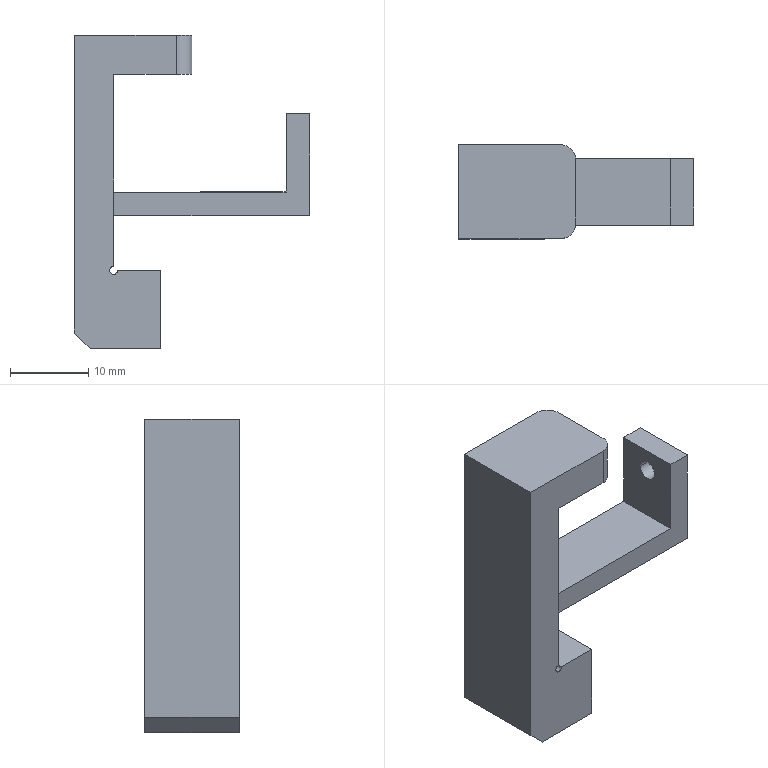Component | SolidWorks | MovingBlock-2 | 1 solid | 24 faces | box 30 x 12 x 40 mm | volume 4558 mm3 | plane 18 | cylinder 6 | commonest cylinder face diameters 2.5 x2 1 x2 4 x2
build123d program:
from build123d import *

# Parameters (mm, degrees)
SKETCH1_W         = 12
SKETCH1_H         = 20
EXTRUDE1_DEPTH    = 5
SKETCH2_W         = 8.5
SKETCH2_H         = 3
EXTRUDE2_DEPTH    = 25
SKETCH3_W         = 12
SKETCH3_H         = 10
EXTRUDE3_DEPTH    = 6
CHAMFER1_SIZE     = 2
SKETCH6_R         = 0.5
EXTRUDE4_DEPTH    = 30.479
SKETCH7_W         = 8.5
SKETCH7_H         = 3
EXTRUDE5_DEPTH    = 10
M3_TAPPED_HOLE1_D = 2.5
SKETCH12_W        = 12
SKETCH12_H        = 5
EXTRUDE8_DEPTH    = 20
SKETCH13_W        = 12
SKETCH13_H        = 5
EXTRUDE9_DEPTH    = 10
FILLET3_R         = 2


with BuildPart() as part:
    # Sketch1 → Extrude1 (new body)
    with BuildSketch(Plane.XY):
        Rectangle(SKETCH1_W, SKETCH1_H)
    extrude(amount=EXTRUDE1_DEPTH)

    # Sketch2 → Extrude2 (add)
    with BuildSketch(Plane(origin=(0, 0, 0), x_dir=(-1, 0, 0), z_dir=(0, 0, -1))):
        with Locations((0, -8.5)):
            Rectangle(SKETCH2_W, SKETCH2_H)
    extrude(amount=EXTRUDE2_DEPTH)

    # Sketch3 → Extrude3 (add)
    with BuildSketch(Plane(origin=(0, 0, 0), x_dir=(-1, 0, 0), z_dir=(0, 0, -1))):
        with Locations((0, 5)):
            Rectangle(SKETCH3_W, SKETCH3_H)
    extrude(amount=EXTRUDE3_DEPTH)

    # Chamfer1
    chamfer1_edges = [part.edges().sort_by_distance(p)[0] for p in [
        (0, 10, 5),
    ]]
    chamfer(chamfer1_edges, length=CHAMFER1_SIZE)

    # Sketch6 → Extrude4 (cut, through all)
    with BuildSketch(Plane.ZY.offset(6)):
        Circle(SKETCH6_R)
    extrude(amount=-EXTRUDE4_DEPTH, mode=Mode.SUBTRACT)

    # Sketch7 → Extrude5 (add)
    with BuildSketch(Plane.XZ.offset(10)):
        with Locations((0, -23.5)):
            Rectangle(SKETCH7_W, SKETCH7_H)
    extrude(amount=EXTRUDE5_DEPTH)

    # M3 Tapped Hole1 (through all)
    with Locations(Plane(origin=(0, 0, -25), x_dir=(-1, 0, 0), z_dir=(0, 0, -1))):
        with Locations((0, -17)):
            Hole(M3_TAPPED_HOLE1_D / 2)

    # Sketch12 → Extrude8 (add)
    with BuildSketch(Plane.XZ.offset(10)):
        with Locations((0, 2.5)):
            Rectangle(SKETCH12_W, SKETCH12_H)
    extrude(amount=EXTRUDE8_DEPTH)

    # Sketch13 → Extrude9 (add)
    with BuildSketch(Plane(origin=(0, 0, 0), x_dir=(-1, 0, 0), z_dir=(0, 0, -1))):
        with Locations((0, -27.5)):
            Rectangle(SKETCH13_W, SKETCH13_H)
    extrude(amount=EXTRUDE9_DEPTH)

    # Fillet3
    fillet3_edges = [part.edges().sort_by_distance(p)[0] for p in [
        (6, -27.5, -10),
        (-6, -27.5, -10),
    ]]
    fillet(fillet3_edges, radius=FILLET3_R)


solid = part.part

# Placed as in the assembly
solid = solid.moved(Location((-89, -31.25, 0), (-90, -90, 0)))
STEP:
#1=CARTESIAN_POINT('',(-2.638,-1.181,0.6693));
#2=VERTEX_POINT('',#1);
#3=CARTESIAN_POINT('',(-2.638,-1.28,0.6693));
#4=VERTEX_POINT('',#3);
#5=CARTESIAN_POINT('',(-2.638,-1.23,0.6693));
#6=DIRECTION('',(1.,0.,0.));
#7=DIRECTION('',(0.,-1.,0.));
#8=AXIS2_PLACEMENT_3D('',#5,#6,#7);
#9=CIRCLE('',#8,0.04921);
#10=EDGE_CURVE('',#2,#4,#9,.T.);
#11=ORIENTED_EDGE('',*,*,#10,.F.);
#12=CARTESIAN_POINT('',(-2.52,-1.181,0.6693));
#13=VERTEX_POINT('',#12);
#14=CARTESIAN_POINT('',(-2.52,-1.181,0.6693));
#15=DIRECTION('',(1.,0.,0.));
#16=VECTOR('',#15,39.37);
#17=LINE('',#14,#16);
#18=EDGE_CURVE('',#2,#13,#17,.T.);
#19=ORIENTED_EDGE('',*,*,#18,.T.);
#20=CARTESIAN_POINT('',(-2.52,-1.28,0.6693));
#21=VERTEX_POINT('',#20);
#22=CARTESIAN_POINT('',(-2.52,-1.23,0.6693));
#23=DIRECTION('',(1.,0.,0.));
#24=DIRECTION('',(0.,-1.,0.));
#25=AXIS2_PLACEMENT_3D('',#22,#23,#24);
#26=CIRCLE('',#25,0.04921);
#27=EDGE_CURVE('',#13,#21,#26,.T.);
#28=ORIENTED_EDGE('',*,*,#27,.T.);
#29=CARTESIAN_POINT('',(-2.52,-1.28,0.6693));
#30=DIRECTION('',(1.,0.,0.));
#31=VECTOR('',#30,39.37);
#32=LINE('',#29,#31);
#33=EDGE_CURVE('',#4,#21,#32,.T.);
#34=ORIENTED_EDGE('',*,*,#33,.F.);
#35=EDGE_LOOP('',(#11,#19,#28,#34));
#36=FACE_OUTER_BOUND('',#35,.T.);
#37=CARTESIAN_POINT('',(-2.52,-1.23,0.6693));
#38=DIRECTION('',(1.,0.,0.));
#39=DIRECTION('',(0.,-1.,0.));
#40=AXIS2_PLACEMENT_3D('',#37,#38,#39);
#41=CYLINDRICAL_SURFACE('',#40,0.04921);
#42=ADVANCED_FACE('',(#36),#41,.F.);
#43=CARTESIAN_POINT('',(-3.524,-0.9941,0.));
#44=VERTEX_POINT('',#43);
#45=CARTESIAN_POINT('',(-3.484,-0.9941,-0.));
#46=VERTEX_POINT('',#45);
#47=CARTESIAN_POINT('',(-3.504,-0.9941,0.));
#48=DIRECTION('',(0.,-1.,0.));
#49=DIRECTION('',(-1.,0.,0.));
#50=AXIS2_PLACEMENT_3D('',#47,#48,#49);
#51=CIRCLE('',#50,0.01969);
#52=EDGE_CURVE('',#44,#46,#51,.T.);
#53=ORIENTED_EDGE('',*,*,#52,.F.);
#54=CARTESIAN_POINT('',(-3.524,-1.467,0.));
#55=VERTEX_POINT('',#54);
#56=CARTESIAN_POINT('',(-3.524,-0.9941,0.));
#57=DIRECTION('',(0.,-1.,0.));
#58=VECTOR('',#57,39.37);
#59=LINE('',#56,#58);
#60=EDGE_CURVE('',#44,#55,#59,.T.);
#61=ORIENTED_EDGE('',*,*,#60,.T.);
#62=CARTESIAN_POINT('',(-3.484,-1.467,-0.));
#63=VERTEX_POINT('',#62);
#64=CARTESIAN_POINT('',(-3.504,-1.467,0.));
#65=DIRECTION('',(0.,-1.,0.));
#66=DIRECTION('',(-1.,0.,0.));
#67=AXIS2_PLACEMENT_3D('',#64,#65,#66);
#68=CIRCLE('',#67,0.01969);
#69=EDGE_CURVE('',#55,#63,#68,.T.);
#70=ORIENTED_EDGE('',*,*,#69,.T.);
#71=CARTESIAN_POINT('',(-3.484,-0.9941,-0.));
#72=DIRECTION('',(0.,-1.,0.));
#73=VECTOR('',#72,39.37);
#74=LINE('',#71,#73);
#75=EDGE_CURVE('',#46,#63,#74,.T.);
#76=ORIENTED_EDGE('',*,*,#75,.F.);
#77=EDGE_LOOP('',(#53,#61,#70,#76));
#78=FACE_OUTER_BOUND('',#77,.T.);
#79=CARTESIAN_POINT('',(-3.504,-0.9941,0.));
#80=DIRECTION('',(0.,-1.,0.));
#81=DIRECTION('',(-1.,0.,0.));
#82=AXIS2_PLACEMENT_3D('',#79,#80,#81);
#83=CYLINDRICAL_SURFACE('',#82,0.01969);
#84=ADVANCED_FACE('',(#78),#83,.F.);
#85=CARTESIAN_POINT('',(-3.504,-1.398,0.3937));
#86=VERTEX_POINT('',#85);
#87=CARTESIAN_POINT('',(-3.504,-1.398,0.2756));
#88=VERTEX_POINT('',#87);
#89=CARTESIAN_POINT('',(-3.504,-1.398,0.3937));
#90=DIRECTION('',(-0.,0.,-1.));
#91=VECTOR('',#90,39.37);
#92=LINE('',#89,#91);
#93=EDGE_CURVE('',#86,#88,#92,.T.);
#94=ORIENTED_EDGE('',*,*,#93,.F.);
#95=CARTESIAN_POINT('',(-3.504,-1.063,0.3937));
#96=VERTEX_POINT('',#95);
#97=CARTESIAN_POINT('',(-3.504,-1.467,0.3937));
#98=DIRECTION('',(0.,1.,-0.));
#99=VECTOR('',#98,39.37);
#100=LINE('',#97,#99);
#101=EDGE_CURVE('',#86,#96,#100,.T.);
#102=ORIENTED_EDGE('',*,*,#101,.T.);
#103=CARTESIAN_POINT('',(-3.504,-1.063,0.2756));
#104=VERTEX_POINT('',#103);
#105=CARTESIAN_POINT('',(-3.504,-1.063,0.3937));
#106=DIRECTION('',(0.,-0.,1.));
#107=VECTOR('',#106,39.37);
#108=LINE('',#105,#107);
#109=EDGE_CURVE('',#104,#96,#108,.T.);
#110=ORIENTED_EDGE('',*,*,#109,.F.);
#111=CARTESIAN_POINT('',(-3.504,-1.063,0.2756));
#112=DIRECTION('',(0.,1.,0.));
#113=VECTOR('',#112,39.37);
#114=LINE('',#111,#113);
#115=EDGE_CURVE('',#88,#104,#114,.T.);
#116=ORIENTED_EDGE('',*,*,#115,.F.);
#117=EDGE_LOOP('',(#94,#102,#110,#116));
#118=FACE_BOUND('',#117,.T.);
#119=CARTESIAN_POINT('',(-3.504,-1.467,0.9843));
#120=VERTEX_POINT('',#119);
#121=CARTESIAN_POINT('',(-3.504,-0.9941,0.9843));
#122=VERTEX_POINT('',#121);
#123=CARTESIAN_POINT('',(-3.504,-0.9941,0.9843));
#124=DIRECTION('',(0.,1.,-0.));
#125=VECTOR('',#124,39.37);
#126=LINE('',#123,#125);
#127=EDGE_CURVE('',#120,#122,#126,.T.);
#128=ORIENTED_EDGE('',*,*,#127,.F.);
#129=CARTESIAN_POINT('',(-3.504,-1.467,0.01969));
#130=VERTEX_POINT('',#129);
#131=CARTESIAN_POINT('',(-3.504,-1.467,0.3937));
#132=DIRECTION('',(0.,-0.,1.));
#133=VECTOR('',#132,39.37);
#134=LINE('',#131,#133);
#135=EDGE_CURVE('',#130,#120,#134,.T.);
#136=ORIENTED_EDGE('',*,*,#135,.F.);
#137=CARTESIAN_POINT('',(-3.504,-0.9941,0.01969));
#138=VERTEX_POINT('',#137);
#139=CARTESIAN_POINT('',(-3.504,-0.9941,0.01969));
#140=DIRECTION('',(0.,1.,-0.));
#141=VECTOR('',#140,39.37);
#142=LINE('',#139,#141);
#143=EDGE_CURVE('',#130,#138,#142,.T.);
#144=ORIENTED_EDGE('',*,*,#143,.T.);
#145=CARTESIAN_POINT('',(-3.504,-0.9941,0.3937));
#146=DIRECTION('',(-0.,0.,-1.));
#147=VECTOR('',#146,39.37);
#148=LINE('',#145,#147);
#149=EDGE_CURVE('',#122,#138,#148,.T.);
#150=ORIENTED_EDGE('',*,*,#149,.F.);
#151=EDGE_LOOP('',(#128,#136,#144,#150));
#152=FACE_OUTER_BOUND('',#151,.T.);
#153=CARTESIAN_POINT('',(-3.504,-1.467,-0.3937));
#154=DIRECTION('',(-1.,-0.,-0.));
#155=DIRECTION('',(0.,1.,-0.));
#156=AXIS2_PLACEMENT_3D('',#153,#154,#155);
#157=PLANE('',#156);
#158=ADVANCED_FACE('',(#118,#152),#157,.F.);
#159=ORIENTED_EDGE('',*,*,#101,.F.);
#160=CARTESIAN_POINT('',(-2.638,-1.398,0.3937));
#161=VERTEX_POINT('',#160);
#162=CARTESIAN_POINT('',(-2.52,-1.398,0.3937));
#163=DIRECTION('',(-1.,0.,-0.));
#164=VECTOR('',#163,39.37);
#165=LINE('',#162,#164);
#166=EDGE_CURVE('',#161,#86,#165,.T.);
#167=ORIENTED_EDGE('',*,*,#166,.F.);
#168=CARTESIAN_POINT('',(-2.638,-1.063,0.3937));
#169=VERTEX_POINT('',#168);
#170=CARTESIAN_POINT('',(-2.638,-1.398,0.3937));
#171=DIRECTION('',(0.,-1.,0.));
#172=VECTOR('',#171,39.37);
#173=LINE('',#170,#172);
#174=EDGE_CURVE('',#169,#161,#173,.T.);
#175=ORIENTED_EDGE('',*,*,#174,.F.);
#176=CARTESIAN_POINT('',(-2.52,-1.063,0.3937));
#177=DIRECTION('',(-1.,0.,-0.));
#178=VECTOR('',#177,39.37);
#179=LINE('',#176,#178);
#180=EDGE_CURVE('',#169,#96,#179,.T.);
#181=ORIENTED_EDGE('',*,*,#180,.T.);
#182=EDGE_LOOP('',(#159,#167,#175,#181));
#183=FACE_OUTER_BOUND('',#182,.T.);
#184=CARTESIAN_POINT('',(-3.701,-0.9941,0.3937));
#185=DIRECTION('',(0.,0.,-1.));
#186=DIRECTION('',(-1.,0.,-0.));
#187=AXIS2_PLACEMENT_3D('',#184,#185,#186);
#188=PLANE('',#187);
#189=ADVANCED_FACE('',(#183),#188,.F.);
#190=CARTESIAN_POINT('',(-3.189,-1.467,0.9843));
#191=VERTEX_POINT('',#190);
#192=CARTESIAN_POINT('',(-3.11,-1.467,0.9843));
#193=DIRECTION('',(-1.,0.,-0.));
#194=VECTOR('',#193,39.37);
#195=LINE('',#192,#194);
#196=EDGE_CURVE('',#191,#120,#195,.T.);
#197=ORIENTED_EDGE('',*,*,#196,.F.);
#198=CARTESIAN_POINT('',(-3.189,-1.467,1.181));
#199=VERTEX_POINT('',#198);
#200=CARTESIAN_POINT('',(-3.189,-1.467,0.3937));
#201=DIRECTION('',(0.,-0.,1.));
#202=VECTOR('',#201,39.37);
#203=LINE('',#200,#202);
#204=EDGE_CURVE('',#191,#199,#203,.T.);
#205=ORIENTED_EDGE('',*,*,#204,.T.);
#206=CARTESIAN_POINT('',(-3.701,-1.467,1.181));
#207=VERTEX_POINT('',#206);
#208=CARTESIAN_POINT('',(-3.701,-1.467,1.181));
#209=DIRECTION('',(1.,0.,0.));
#210=VECTOR('',#209,39.37);
#211=LINE('',#208,#210);
#212=EDGE_CURVE('',#207,#199,#211,.T.);
#213=ORIENTED_EDGE('',*,*,#212,.F.);
#214=CARTESIAN_POINT('',(-3.701,-1.467,-0.315));
#215=VERTEX_POINT('',#214);
#216=CARTESIAN_POINT('',(-3.701,-1.467,0.3937));
#217=DIRECTION('',(0.,-0.,1.));
#218=VECTOR('',#217,39.37);
#219=LINE('',#216,#218);
#220=EDGE_CURVE('',#215,#207,#219,.T.);
#221=ORIENTED_EDGE('',*,*,#220,.F.);
#222=CARTESIAN_POINT('',(-3.622,-1.467,-0.3937));
#223=VERTEX_POINT('',#222);
#224=CARTESIAN_POINT('',(-3.701,-1.467,-0.315));
#225=DIRECTION('',(0.7071,0.,-0.7071));
#226=VECTOR('',#225,39.37);
#227=LINE('',#224,#226);
#228=EDGE_CURVE('',#215,#223,#227,.T.);
#229=ORIENTED_EDGE('',*,*,#228,.T.);
#230=CARTESIAN_POINT('',(-3.268,-1.467,-0.3937));
#231=VERTEX_POINT('',#230);
#232=CARTESIAN_POINT('',(-3.701,-1.467,-0.3937));
#233=DIRECTION('',(1.,0.,0.));
#234=VECTOR('',#233,39.37);
#235=LINE('',#232,#234);
#236=EDGE_CURVE('',#223,#231,#235,.T.);
#237=ORIENTED_EDGE('',*,*,#236,.T.);
#238=CARTESIAN_POINT('',(-3.268,-1.467,-0.));
#239=VERTEX_POINT('',#238);
#240=CARTESIAN_POINT('',(-3.268,-1.467,-0.3937));
#241=DIRECTION('',(-0.,0.,-1.));
#242=VECTOR('',#241,39.37);
#243=LINE('',#240,#242);
#244=EDGE_CURVE('',#239,#231,#243,.T.);
#245=ORIENTED_EDGE('',*,*,#244,.F.);
#246=CARTESIAN_POINT('',(-3.268,-1.467,-0.));
#247=DIRECTION('',(-1.,0.,-0.));
#248=VECTOR('',#247,39.37);
#249=LINE('',#246,#248);
#250=EDGE_CURVE('',#239,#63,#249,.T.);
#251=ORIENTED_EDGE('',*,*,#250,.T.);
#252=ORIENTED_EDGE('',*,*,#69,.F.);
#253=CARTESIAN_POINT('',(-3.504,-1.467,0.));
#254=DIRECTION('',(0.,-1.,0.));
#255=DIRECTION('',(-1.,0.,0.));
#256=AXIS2_PLACEMENT_3D('',#253,#254,#255);
#257=CIRCLE('',#256,0.01969);
#258=EDGE_CURVE('',#130,#55,#257,.T.);
#259=ORIENTED_EDGE('',*,*,#258,.F.);
#260=ORIENTED_EDGE('',*,*,#135,.T.);
#261=EDGE_LOOP('',(#197,#205,#213,#221,#229,#237,#245,#251,#252,#259,#260));
#262=FACE_OUTER_BOUND('',#261,.T.);
#263=CARTESIAN_POINT('',(-3.701,-1.467,0.3937));
#264=DIRECTION('',(0.,1.,-0.));
#265=DIRECTION('',(1.,0.,0.));
#266=AXIS2_PLACEMENT_3D('',#263,#264,#265);
#267=PLANE('',#266);
#268=ADVANCED_FACE('',(#262),#267,.F.);
#269=CARTESIAN_POINT('',(-3.189,-0.9941,1.181));
#270=VERTEX_POINT('',#269);
#271=CARTESIAN_POINT('',(-3.701,-0.9941,1.181));
#272=VERTEX_POINT('',#271);
#273=CARTESIAN_POINT('',(-3.701,-0.9941,1.181));
#274=DIRECTION('',(-1.,0.,-0.));
#275=VECTOR('',#274,39.37);
#276=LINE('',#273,#275);
#277=EDGE_CURVE('',#270,#272,#276,.T.);
#278=ORIENTED_EDGE('',*,*,#277,.F.);
#279=CARTESIAN_POINT('',(-3.189,-0.9941,0.9843));
#280=VERTEX_POINT('',#279);
#281=CARTESIAN_POINT('',(-3.189,-0.9941,0.3937));
#282=DIRECTION('',(-0.,0.,-1.));
#283=VECTOR('',#282,39.37);
#284=LINE('',#281,#283);
#285=EDGE_CURVE('',#270,#280,#284,.T.);
#286=ORIENTED_EDGE('',*,*,#285,.T.);
#287=CARTESIAN_POINT('',(-3.11,-0.9941,0.9843));
#288=DIRECTION('',(-1.,0.,-0.));
#289=VECTOR('',#288,39.37);
#290=LINE('',#287,#289);
#291=EDGE_CURVE('',#280,#122,#290,.T.);
#292=ORIENTED_EDGE('',*,*,#291,.T.);
#293=ORIENTED_EDGE('',*,*,#149,.T.);
#294=CARTESIAN_POINT('',(-3.504,-0.9941,0.));
#295=DIRECTION('',(0.,-1.,0.));
#296=DIRECTION('',(-1.,0.,0.));
#297=AXIS2_PLACEMENT_3D('',#294,#295,#296);
#298=CIRCLE('',#297,0.01969);
#299=EDGE_CURVE('',#138,#44,#298,.T.);
#300=ORIENTED_EDGE('',*,*,#299,.T.);
#301=ORIENTED_EDGE('',*,*,#52,.T.);
#302=CARTESIAN_POINT('',(-3.268,-0.9941,-0.));
#303=VERTEX_POINT('',#302);
#304=CARTESIAN_POINT('',(-3.268,-0.9941,-0.));
#305=DIRECTION('',(-1.,0.,-0.));
#306=VECTOR('',#305,39.37);
#307=LINE('',#304,#306);
#308=EDGE_CURVE('',#303,#46,#307,.T.);
#309=ORIENTED_EDGE('',*,*,#308,.F.);
#310=CARTESIAN_POINT('',(-3.268,-0.9941,-0.3937));
#311=VERTEX_POINT('',#310);
#312=CARTESIAN_POINT('',(-3.268,-0.9941,-0.3937));
#313=DIRECTION('',(0.,-0.,1.));
#314=VECTOR('',#313,39.37);
#315=LINE('',#312,#314);
#316=EDGE_CURVE('',#311,#303,#315,.T.);
#317=ORIENTED_EDGE('',*,*,#316,.F.);
#318=CARTESIAN_POINT('',(-3.622,-0.9941,-0.3937));
#319=VERTEX_POINT('',#318);
#320=CARTESIAN_POINT('',(-3.701,-0.9941,-0.3937));
#321=DIRECTION('',(1.,0.,0.));
#322=VECTOR('',#321,39.37);
#323=LINE('',#320,#322);
#324=EDGE_CURVE('',#319,#311,#323,.T.);
#325=ORIENTED_EDGE('',*,*,#324,.F.);
#326=CARTESIAN_POINT('',(-3.701,-0.9941,-0.315));
#327=VERTEX_POINT('',#326);
#328=CARTESIAN_POINT('',(-3.701,-0.9941,-0.315));
#329=DIRECTION('',(-0.7071,-0.,0.7071));
#330=VECTOR('',#329,39.37);
#331=LINE('',#328,#330);
#332=EDGE_CURVE('',#319,#327,#331,.T.);
#333=ORIENTED_EDGE('',*,*,#332,.T.);
#334=CARTESIAN_POINT('',(-3.701,-0.9941,0.3937));
#335=DIRECTION('',(-0.,0.,-1.));
#336=VECTOR('',#335,39.37);
#337=LINE('',#334,#336);
#338=EDGE_CURVE('',#272,#327,#337,.T.);
#339=ORIENTED_EDGE('',*,*,#338,.F.);
#340=EDGE_LOOP('',(#278,#286,#292,#293,#300,#301,#309,#317,#325,#333,#339));
#341=FACE_OUTER_BOUND('',#340,.T.);
#342=CARTESIAN_POINT('',(-3.701,-0.9941,0.3937));
#343=DIRECTION('',(-0.,-1.,0.));
#344=DIRECTION('',(-1.,0.,-0.));
#345=AXIS2_PLACEMENT_3D('',#342,#343,#344);
#346=PLANE('',#345);
#347=ADVANCED_FACE('',(#341),#346,.F.);
#348=ORIENTED_EDGE('',*,*,#236,.F.);
#349=CARTESIAN_POINT('',(-3.622,-0.9941,-0.3937));
#350=DIRECTION('',(-0.,1.,-0.));
#351=VECTOR('',#350,39.37);
#352=LINE('',#349,#351);
#353=EDGE_CURVE('',#223,#319,#352,.T.);
#354=ORIENTED_EDGE('',*,*,#353,.T.);
#355=ORIENTED_EDGE('',*,*,#324,.T.);
#356=CARTESIAN_POINT('',(-3.268,-0.9941,-0.3937));
#357=DIRECTION('',(0.,1.,-0.));
#358=VECTOR('',#357,39.37);
#359=LINE('',#356,#358);
#360=EDGE_CURVE('',#231,#311,#359,.T.);
#361=ORIENTED_EDGE('',*,*,#360,.F.);
#362=EDGE_LOOP('',(#348,#354,#355,#361));
#363=FACE_OUTER_BOUND('',#362,.T.);
#364=CARTESIAN_POINT('',(-3.701,-0.9941,-0.3937));
#365=DIRECTION('',(0.,0.,1.));
#366=DIRECTION('',(-0.,1.,-0.));
#367=AXIS2_PLACEMENT_3D('',#364,#365,#366);
#368=PLANE('',#367);
#369=ADVANCED_FACE('',(#363),#368,.F.);
#370=ORIENTED_EDGE('',*,*,#338,.T.);
#371=CARTESIAN_POINT('',(-3.701,-1.467,-0.315));
#372=DIRECTION('',(0.,-1.,0.));
#373=VECTOR('',#372,39.37);
#374=LINE('',#371,#373);
#375=EDGE_CURVE('',#327,#215,#374,.T.);
#376=ORIENTED_EDGE('',*,*,#375,.T.);
#377=ORIENTED_EDGE('',*,*,#220,.T.);
#378=CARTESIAN_POINT('',(-3.701,-1.467,1.181));
#379=DIRECTION('',(0.,-1.,0.));
#380=VECTOR('',#379,39.37);
#381=LINE('',#378,#380);
#382=EDGE_CURVE('',#272,#207,#381,.T.);
#383=ORIENTED_EDGE('',*,*,#382,.F.);
#384=EDGE_LOOP('',(#370,#376,#377,#383));
#385=FACE_OUTER_BOUND('',#384,.T.);
#386=CARTESIAN_POINT('',(-3.701,-1.467,-0.3937));
#387=DIRECTION('',(-1.,-0.,-0.));
#388=DIRECTION('',(0.,1.,-0.));
#389=AXIS2_PLACEMENT_3D('',#386,#387,#388);
#390=PLANE('',#389);
#391=ADVANCED_FACE('',(#385),#390,.T.);
#392=ORIENTED_EDGE('',*,*,#109,.T.);
#393=ORIENTED_EDGE('',*,*,#180,.F.);
#394=CARTESIAN_POINT('',(-2.638,-1.063,0.7874));
#395=VERTEX_POINT('',#394);
#396=CARTESIAN_POINT('',(-2.638,-1.063,0.7874));
#397=DIRECTION('',(-0.,0.,-1.));
#398=VECTOR('',#397,39.37);
#399=LINE('',#396,#398);
#400=EDGE_CURVE('',#395,#169,#399,.T.);
#401=ORIENTED_EDGE('',*,*,#400,.F.);
#402=CARTESIAN_POINT('',(-2.52,-1.063,0.7874));
#403=VERTEX_POINT('',#402);
#404=CARTESIAN_POINT('',(-2.52,-1.063,0.7874));
#405=DIRECTION('',(-1.,0.,-0.));
#406=VECTOR('',#405,39.37);
#407=LINE('',#404,#406);
#408=EDGE_CURVE('',#403,#395,#407,.T.);
#409=ORIENTED_EDGE('',*,*,#408,.F.);
#410=CARTESIAN_POINT('',(-2.52,-1.063,0.2756));
#411=VERTEX_POINT('',#410);
#412=CARTESIAN_POINT('',(-2.52,-1.063,0.3937));
#413=DIRECTION('',(0.,-0.,1.));
#414=VECTOR('',#413,39.37);
#415=LINE('',#412,#414);
#416=EDGE_CURVE('',#411,#403,#415,.T.);
#417=ORIENTED_EDGE('',*,*,#416,.F.);
#418=CARTESIAN_POINT('',(-2.52,-1.063,0.2756));
#419=DIRECTION('',(-1.,0.,-0.));
#420=VECTOR('',#419,39.37);
#421=LINE('',#418,#420);
#422=EDGE_CURVE('',#411,#104,#421,.T.);
#423=ORIENTED_EDGE('',*,*,#422,.T.);
#424=EDGE_LOOP('',(#392,#393,#401,#409,#417,#423));
#425=FACE_OUTER_BOUND('',#424,.T.);
#426=CARTESIAN_POINT('',(-2.52,-1.063,0.3937));
#427=DIRECTION('',(-0.,-1.,0.));
#428=DIRECTION('',(-1.,0.,-0.));
#429=AXIS2_PLACEMENT_3D('',#426,#427,#428);
#430=PLANE('',#429);
#431=ADVANCED_FACE('',(#425),#430,.F.);
#432=ORIENTED_EDGE('',*,*,#93,.T.);
#433=CARTESIAN_POINT('',(-2.52,-1.398,0.2756));
#434=VERTEX_POINT('',#433);
#435=CARTESIAN_POINT('',(-2.52,-1.398,0.2756));
#436=DIRECTION('',(-1.,0.,-0.));
#437=VECTOR('',#436,39.37);
#438=LINE('',#435,#437);
#439=EDGE_CURVE('',#434,#88,#438,.T.);
#440=ORIENTED_EDGE('',*,*,#439,.F.);
#441=CARTESIAN_POINT('',(-2.52,-1.398,0.7874));
#442=VERTEX_POINT('',#441);
#443=CARTESIAN_POINT('',(-2.52,-1.398,0.3937));
#444=DIRECTION('',(-0.,0.,-1.));
#445=VECTOR('',#444,39.37);
#446=LINE('',#443,#445);
#447=EDGE_CURVE('',#442,#434,#446,.T.);
#448=ORIENTED_EDGE('',*,*,#447,.F.);
#449=CARTESIAN_POINT('',(-2.638,-1.398,0.7874));
#450=VERTEX_POINT('',#449);
#451=CARTESIAN_POINT('',(-2.52,-1.398,0.7874));
#452=DIRECTION('',(1.,0.,0.));
#453=VECTOR('',#452,39.37);
#454=LINE('',#451,#453);
#455=EDGE_CURVE('',#450,#442,#454,.T.);
#456=ORIENTED_EDGE('',*,*,#455,.F.);
#457=CARTESIAN_POINT('',(-2.638,-1.398,0.7874));
#458=DIRECTION('',(-0.,0.,-1.));
#459=VECTOR('',#458,39.37);
#460=LINE('',#457,#459);
#461=EDGE_CURVE('',#450,#161,#460,.T.);
#462=ORIENTED_EDGE('',*,*,#461,.T.);
#463=ORIENTED_EDGE('',*,*,#166,.T.);
#464=EDGE_LOOP('',(#432,#440,#448,#456,#462,#463));
#465=FACE_OUTER_BOUND('',#464,.T.);
#466=CARTESIAN_POINT('',(-2.52,-1.398,0.3937));
#467=DIRECTION('',(0.,1.,-0.));
#468=DIRECTION('',(1.,0.,0.));
#469=AXIS2_PLACEMENT_3D('',#466,#467,#468);
#470=PLANE('',#469);
#471=ADVANCED_FACE('',(#465),#470,.F.);
#472=ORIENTED_EDGE('',*,*,#115,.T.);
#473=ORIENTED_EDGE('',*,*,#422,.F.);
#474=CARTESIAN_POINT('',(-2.52,-1.063,0.2756));
#475=DIRECTION('',(0.,1.,0.));
#476=VECTOR('',#475,39.37);
#477=LINE('',#474,#476);
#478=EDGE_CURVE('',#434,#411,#477,.T.);
#479=ORIENTED_EDGE('',*,*,#478,.F.);
#480=ORIENTED_EDGE('',*,*,#439,.T.);
#481=EDGE_LOOP('',(#472,#473,#479,#480));
#482=FACE_OUTER_BOUND('',#481,.T.);
#483=CARTESIAN_POINT('',(-2.52,-1.063,0.2756));
#484=DIRECTION('',(0.,-0.,1.));
#485=DIRECTION('',(0.,1.,0.));
#486=AXIS2_PLACEMENT_3D('',#483,#484,#485);
#487=PLANE('',#486);
#488=ADVANCED_FACE('',(#482),#487,.F.);
#489=CARTESIAN_POINT('',(-2.52,-1.23,0.6693));
#490=DIRECTION('',(1.,0.,0.));
#491=DIRECTION('',(0.,-1.,0.));
#492=AXIS2_PLACEMENT_3D('',#489,#490,#491);
#493=CIRCLE('',#492,0.04921);
#494=EDGE_CURVE('',#21,#13,#493,.T.);
#495=ORIENTED_EDGE('',*,*,#494,.F.);
#496=ORIENTED_EDGE('',*,*,#27,.F.);
#497=EDGE_LOOP('',(#495,#496));
#498=FACE_BOUND('',#497,.T.);
#499=ORIENTED_EDGE('',*,*,#416,.T.);
#500=CARTESIAN_POINT('',(-2.52,-1.398,0.7874));
#501=DIRECTION('',(0.,1.,-0.));
#502=VECTOR('',#501,39.37);
#503=LINE('',#500,#502);
#504=EDGE_CURVE('',#442,#403,#503,.T.);
#505=ORIENTED_EDGE('',*,*,#504,.F.);
#506=ORIENTED_EDGE('',*,*,#447,.T.);
#507=ORIENTED_EDGE('',*,*,#478,.T.);
#508=EDGE_LOOP('',(#499,#505,#506,#507));
#509=FACE_OUTER_BOUND('',#508,.T.);
#510=CARTESIAN_POINT('',(-2.52,-1.063,0.2756));
#511=DIRECTION('',(-1.,-0.,-0.));
#512=DIRECTION('',(0.,1.,-0.));
#513=AXIS2_PLACEMENT_3D('',#510,#511,#512);
#514=PLANE('',#513);
#515=ADVANCED_FACE('',(#498,#509),#514,.F.);
#516=ORIENTED_EDGE('',*,*,#308,.T.);
#517=ORIENTED_EDGE('',*,*,#75,.T.);
#518=ORIENTED_EDGE('',*,*,#250,.F.);
#519=CARTESIAN_POINT('',(-3.268,-0.9941,-0.));
#520=DIRECTION('',(0.,-1.,0.));
#521=VECTOR('',#520,39.37);
#522=LINE('',#519,#521);
#523=EDGE_CURVE('',#303,#239,#522,.T.);
#524=ORIENTED_EDGE('',*,*,#523,.F.);
#525=EDGE_LOOP('',(#516,#517,#518,#524));
#526=FACE_OUTER_BOUND('',#525,.T.);
#527=CARTESIAN_POINT('',(-3.268,-0.9941,-0.));
#528=DIRECTION('',(0.,0.,-1.));
#529=DIRECTION('',(-1.,0.,-0.));
#530=AXIS2_PLACEMENT_3D('',#527,#528,#529);
#531=PLANE('',#530);
#532=ADVANCED_FACE('',(#526),#531,.F.);
#533=ORIENTED_EDGE('',*,*,#316,.T.);
#534=ORIENTED_EDGE('',*,*,#523,.T.);
#535=ORIENTED_EDGE('',*,*,#244,.T.);
#536=ORIENTED_EDGE('',*,*,#360,.T.);
#537=EDGE_LOOP('',(#533,#534,#535,#536));
#538=FACE_OUTER_BOUND('',#537,.T.);
#539=CARTESIAN_POINT('',(-3.268,-0.9941,-0.));
#540=DIRECTION('',(1.,0.,0.));
#541=DIRECTION('',(0.,-1.,0.));
#542=AXIS2_PLACEMENT_3D('',#539,#540,#541);
#543=PLANE('',#542);
#544=ADVANCED_FACE('',(#538),#543,.T.);
#545=ORIENTED_EDGE('',*,*,#332,.F.);
#546=ORIENTED_EDGE('',*,*,#353,.F.);
#547=ORIENTED_EDGE('',*,*,#228,.F.);
#548=ORIENTED_EDGE('',*,*,#375,.F.);
#549=EDGE_LOOP('',(#545,#546,#547,#548));
#550=FACE_OUTER_BOUND('',#549,.T.);
#551=CARTESIAN_POINT('',(-3.701,-1.467,-0.315));
#552=DIRECTION('',(-0.7071,-0.,-0.7071));
#553=DIRECTION('',(-0.7071,-0.,0.7071));
#554=AXIS2_PLACEMENT_3D('',#551,#552,#553);
#555=PLANE('',#554);
#556=ADVANCED_FACE('',(#550),#555,.T.);
#557=ORIENTED_EDGE('',*,*,#60,.F.);
#558=ORIENTED_EDGE('',*,*,#299,.F.);
#559=ORIENTED_EDGE('',*,*,#143,.F.);
#560=ORIENTED_EDGE('',*,*,#258,.T.);
#561=EDGE_LOOP('',(#557,#558,#559,#560));
#562=FACE_OUTER_BOUND('',#561,.T.);
#563=CARTESIAN_POINT('',(-3.504,-0.9941,0.));
#564=DIRECTION('',(0.,-1.,0.));
#565=DIRECTION('',(-1.,0.,0.));
#566=AXIS2_PLACEMENT_3D('',#563,#564,#565);
#567=CYLINDRICAL_SURFACE('',#566,0.01969);
#568=ADVANCED_FACE('',(#562),#567,.F.);
#569=CARTESIAN_POINT('',(-2.638,-1.23,0.6693));
#570=DIRECTION('',(1.,0.,0.));
#571=DIRECTION('',(0.,-1.,0.));
#572=AXIS2_PLACEMENT_3D('',#569,#570,#571);
#573=CIRCLE('',#572,0.04921);
#574=EDGE_CURVE('',#4,#2,#573,.T.);
#575=ORIENTED_EDGE('',*,*,#574,.T.);
#576=ORIENTED_EDGE('',*,*,#10,.T.);
#577=EDGE_LOOP('',(#575,#576));
#578=FACE_BOUND('',#577,.T.);
#579=ORIENTED_EDGE('',*,*,#174,.T.);
#580=ORIENTED_EDGE('',*,*,#461,.F.);
#581=CARTESIAN_POINT('',(-2.638,-1.398,0.7874));
#582=DIRECTION('',(0.,-1.,0.));
#583=VECTOR('',#582,39.37);
#584=LINE('',#581,#583);
#585=EDGE_CURVE('',#395,#450,#584,.T.);
#586=ORIENTED_EDGE('',*,*,#585,.F.);
#587=ORIENTED_EDGE('',*,*,#400,.T.);
#588=EDGE_LOOP('',(#579,#580,#586,#587));
#589=FACE_OUTER_BOUND('',#588,.T.);
#590=CARTESIAN_POINT('',(-2.638,-1.398,0.7874));
#591=DIRECTION('',(1.,0.,0.));
#592=DIRECTION('',(0.,-1.,0.));
#593=AXIS2_PLACEMENT_3D('',#590,#591,#592);
#594=PLANE('',#593);
#595=ADVANCED_FACE('',(#578,#589),#594,.F.);
#596=ORIENTED_EDGE('',*,*,#455,.T.);
#597=ORIENTED_EDGE('',*,*,#504,.T.);
#598=ORIENTED_EDGE('',*,*,#408,.T.);
#599=ORIENTED_EDGE('',*,*,#585,.T.);
#600=EDGE_LOOP('',(#596,#597,#598,#599));
#601=FACE_OUTER_BOUND('',#600,.T.);
#602=CARTESIAN_POINT('',(-2.638,-1.398,0.7874));
#603=DIRECTION('',(0.,0.,-1.));
#604=DIRECTION('',(-1.,0.,-0.));
#605=AXIS2_PLACEMENT_3D('',#602,#603,#604);
#606=PLANE('',#605);
#607=ADVANCED_FACE('',(#601),#606,.F.);
#608=ORIENTED_EDGE('',*,*,#18,.F.);
#609=ORIENTED_EDGE('',*,*,#574,.F.);
#610=ORIENTED_EDGE('',*,*,#33,.T.);
#611=ORIENTED_EDGE('',*,*,#494,.T.);
#612=EDGE_LOOP('',(#608,#609,#610,#611));
#613=FACE_OUTER_BOUND('',#612,.T.);
#614=CARTESIAN_POINT('',(-2.52,-1.23,0.6693));
#615=DIRECTION('',(1.,0.,0.));
#616=DIRECTION('',(0.,-1.,0.));
#617=AXIS2_PLACEMENT_3D('',#614,#615,#616);
#618=CYLINDRICAL_SURFACE('',#617,0.04921);
#619=ADVANCED_FACE('',(#613),#618,.F.);
#620=ORIENTED_EDGE('',*,*,#212,.T.);
#621=CARTESIAN_POINT('',(-3.11,-1.388,1.181));
#622=VERTEX_POINT('',#621);
#623=CARTESIAN_POINT('',(-3.189,-1.388,1.181));
#624=DIRECTION('',(0.,-0.,1.));
#625=DIRECTION('',(1.,0.,0.));
#626=AXIS2_PLACEMENT_3D('',#623,#624,#625);
#627=CIRCLE('',#626,0.07874);
#628=EDGE_CURVE('',#199,#622,#627,.T.);
#629=ORIENTED_EDGE('',*,*,#628,.T.);
#630=CARTESIAN_POINT('',(-3.11,-1.073,1.181));
#631=VERTEX_POINT('',#630);
#632=CARTESIAN_POINT('',(-3.11,-0.9941,1.181));
#633=DIRECTION('',(0.,-1.,0.));
#634=VECTOR('',#633,39.37);
#635=LINE('',#632,#634);
#636=EDGE_CURVE('',#631,#622,#635,.T.);
#637=ORIENTED_EDGE('',*,*,#636,.F.);
#638=CARTESIAN_POINT('',(-3.189,-1.073,1.181));
#639=DIRECTION('',(0.,-0.,1.));
#640=DIRECTION('',(1.,0.,0.));
#641=AXIS2_PLACEMENT_3D('',#638,#639,#640);
#642=CIRCLE('',#641,0.07874);
#643=EDGE_CURVE('',#631,#270,#642,.T.);
#644=ORIENTED_EDGE('',*,*,#643,.T.);
#645=ORIENTED_EDGE('',*,*,#277,.T.);
#646=ORIENTED_EDGE('',*,*,#382,.T.);
#647=EDGE_LOOP('',(#620,#629,#637,#644,#645,#646));
#648=FACE_OUTER_BOUND('',#647,.T.);
#649=CARTESIAN_POINT('',(-3.504,-1.467,1.181));
#650=DIRECTION('',(-0.,-0.,1.));
#651=DIRECTION('',(1.,0.,0.));
#652=AXIS2_PLACEMENT_3D('',#649,#650,#651);
#653=PLANE('',#652);
#654=ADVANCED_FACE('',(#648),#653,.T.);
#655=CARTESIAN_POINT('',(-3.11,-1.388,0.9843));
#656=VERTEX_POINT('',#655);
#657=CARTESIAN_POINT('',(-3.11,-1.073,0.9843));
#658=VERTEX_POINT('',#657);
#659=CARTESIAN_POINT('',(-3.11,-0.9941,0.9843));
#660=DIRECTION('',(0.,1.,-0.));
#661=VECTOR('',#660,39.37);
#662=LINE('',#659,#661);
#663=EDGE_CURVE('',#656,#658,#662,.T.);
#664=ORIENTED_EDGE('',*,*,#663,.F.);
#665=CARTESIAN_POINT('',(-3.189,-1.388,0.9843));
#666=DIRECTION('',(-0.,0.,-1.));
#667=DIRECTION('',(1.,0.,0.));
#668=AXIS2_PLACEMENT_3D('',#665,#666,#667);
#669=CIRCLE('',#668,0.07874);
#670=EDGE_CURVE('',#656,#191,#669,.T.);
#671=ORIENTED_EDGE('',*,*,#670,.T.);
#672=ORIENTED_EDGE('',*,*,#196,.T.);
#673=ORIENTED_EDGE('',*,*,#127,.T.);
#674=ORIENTED_EDGE('',*,*,#291,.F.);
#675=CARTESIAN_POINT('',(-3.189,-1.073,0.9843));
#676=DIRECTION('',(-0.,0.,-1.));
#677=DIRECTION('',(1.,0.,0.));
#678=AXIS2_PLACEMENT_3D('',#675,#676,#677);
#679=CIRCLE('',#678,0.07874);
#680=EDGE_CURVE('',#280,#658,#679,.T.);
#681=ORIENTED_EDGE('',*,*,#680,.T.);
#682=EDGE_LOOP('',(#664,#671,#672,#673,#674,#681));
#683=FACE_OUTER_BOUND('',#682,.T.);
#684=CARTESIAN_POINT('',(-3.11,-0.9941,0.9843));
#685=DIRECTION('',(-0.,-0.,1.));
#686=DIRECTION('',(1.,0.,0.));
#687=AXIS2_PLACEMENT_3D('',#684,#685,#686);
#688=PLANE('',#687);
#689=ADVANCED_FACE('',(#683),#688,.F.);
#690=ORIENTED_EDGE('',*,*,#636,.T.);
#691=CARTESIAN_POINT('',(-3.11,-1.388,0.9843));
#692=DIRECTION('',(-0.,0.,-1.));
#693=VECTOR('',#692,39.37);
#694=LINE('',#691,#693);
#695=EDGE_CURVE('',#622,#656,#694,.T.);
#696=ORIENTED_EDGE('',*,*,#695,.T.);
#697=ORIENTED_EDGE('',*,*,#663,.T.);
#698=CARTESIAN_POINT('',(-3.11,-1.073,0.9843));
#699=DIRECTION('',(0.,-0.,1.));
#700=VECTOR('',#699,39.37);
#701=LINE('',#698,#700);
#702=EDGE_CURVE('',#658,#631,#701,.T.);
#703=ORIENTED_EDGE('',*,*,#702,.T.);
#704=EDGE_LOOP('',(#690,#696,#697,#703));
#705=FACE_OUTER_BOUND('',#704,.T.);
#706=CARTESIAN_POINT('',(-3.11,-0.9941,0.9843));
#707=DIRECTION('',(-1.,-0.,-0.));
#708=DIRECTION('',(0.,1.,-0.));
#709=AXIS2_PLACEMENT_3D('',#706,#707,#708);
#710=PLANE('',#709);
#711=ADVANCED_FACE('',(#705),#710,.F.);
#712=ORIENTED_EDGE('',*,*,#628,.F.);
#713=ORIENTED_EDGE('',*,*,#204,.F.);
#714=ORIENTED_EDGE('',*,*,#670,.F.);
#715=ORIENTED_EDGE('',*,*,#695,.F.);
#716=EDGE_LOOP('',(#712,#713,#714,#715));
#717=FACE_OUTER_BOUND('',#716,.T.);
#718=CARTESIAN_POINT('',(-3.189,-1.388,0.9843));
#719=DIRECTION('',(-0.,0.,-1.));
#720=DIRECTION('',(-1.,0.,0.));
#721=AXIS2_PLACEMENT_3D('',#718,#719,#720);
#722=CYLINDRICAL_SURFACE('',#721,0.07874);
#723=ADVANCED_FACE('',(#717),#722,.T.);
#724=ORIENTED_EDGE('',*,*,#680,.F.);
#725=ORIENTED_EDGE('',*,*,#285,.F.);
#726=ORIENTED_EDGE('',*,*,#643,.F.);
#727=ORIENTED_EDGE('',*,*,#702,.F.);
#728=EDGE_LOOP('',(#724,#725,#726,#727));
#729=FACE_OUTER_BOUND('',#728,.T.);
#730=CARTESIAN_POINT('',(-3.189,-1.073,0.9843));
#731=DIRECTION('',(0.,-0.,1.));
#732=DIRECTION('',(1.,0.,0.));
#733=AXIS2_PLACEMENT_3D('',#730,#731,#732);
#734=CYLINDRICAL_SURFACE('',#733,0.07874);
#735=ADVANCED_FACE('',(#729),#734,.T.);
#736=CLOSED_SHELL('',(#42,#84,#158,#189,#268,#347,#369,#391,#431,#471,#488,#515,#532,#544,#556,#568,#595,#607,#619,#654,#689,#711,#723,#735));
#737=MANIFOLD_SOLID_BREP('',#736);
#738=CARTESIAN_POINT('',(0.,0.,0.));
#739=DIRECTION('',(0.,0.,1.));
#740=DIRECTION('',(1.,0.,0.));
#741=AXIS2_PLACEMENT_3D('',#738,#739,#740);
#742=(LENGTH_UNIT()NAMED_UNIT(*)SI_UNIT($,.METRE.));
#743=LENGTH_MEASURE_WITH_UNIT(LENGTH_MEASURE(0.0254),#742);
#744=DIMENSIONAL_EXPONENTS(1.,0.,0.,0.,0.,0.,0.);
#745=(CONVERSION_BASED_UNIT('',#743)LENGTH_UNIT()NAMED_UNIT(#744));
#746=UNCERTAINTY_MEASURE_WITH_UNIT(LENGTH_MEASURE(0.00001),#745,'','');
#747=(NAMED_UNIT(*)PLANE_ANGLE_UNIT()SI_UNIT($,.RADIAN.));
#748=(NAMED_UNIT(*)SI_UNIT($,.STERADIAN.)SOLID_ANGLE_UNIT());
#749=(GEOMETRIC_REPRESENTATION_CONTEXT(3)GLOBAL_UNCERTAINTY_ASSIGNED_CONTEXT((#746))GLOBAL_UNIT_ASSIGNED_CONTEXT((#745,#747,#748))REPRESENTATION_CONTEXT('',''));
#750=ADVANCED_BREP_SHAPE_REPRESENTATION('',(#737,#741),#749);
#751=COLOUR_RGB('',0.7922,0.8196,0.9333);
#752=FILL_AREA_STYLE_COLOUR('',#751);
#753=FILL_AREA_STYLE('',(#752));
#754=SURFACE_STYLE_FILL_AREA(#753);
#755=SURFACE_SIDE_STYLE('',(#754));
#756=SURFACE_STYLE_USAGE(.BOTH.,#755);
#757=PRESENTATION_STYLE_ASSIGNMENT((#756));
#758=STYLED_ITEM('',(#757),#737);
#759=(LENGTH_UNIT()NAMED_UNIT(*)SI_UNIT($,.METRE.));
#760=LENGTH_MEASURE_WITH_UNIT(LENGTH_MEASURE(0.0254),#759);
#761=DIMENSIONAL_EXPONENTS(1.,0.,0.,0.,0.,0.,0.);
#762=(CONVERSION_BASED_UNIT('',#760)LENGTH_UNIT()NAMED_UNIT(#761));
#763=UNCERTAINTY_MEASURE_WITH_UNIT(LENGTH_MEASURE(0.00001),#762,'','');
#764=(NAMED_UNIT(*)PLANE_ANGLE_UNIT()SI_UNIT($,.RADIAN.));
#765=(NAMED_UNIT(*)SI_UNIT($,.STERADIAN.)SOLID_ANGLE_UNIT());
#766=(GEOMETRIC_REPRESENTATION_CONTEXT(3)GLOBAL_UNCERTAINTY_ASSIGNED_CONTEXT((#763))GLOBAL_UNIT_ASSIGNED_CONTEXT((#762,#764,#765))REPRESENTATION_CONTEXT('',''));
#767=MECHANICAL_DESIGN_GEOMETRIC_PRESENTATION_REPRESENTATION('',(#758),#766);
#768=PRESENTATION_LAYER_ASSIGNMENT('','',(#758));